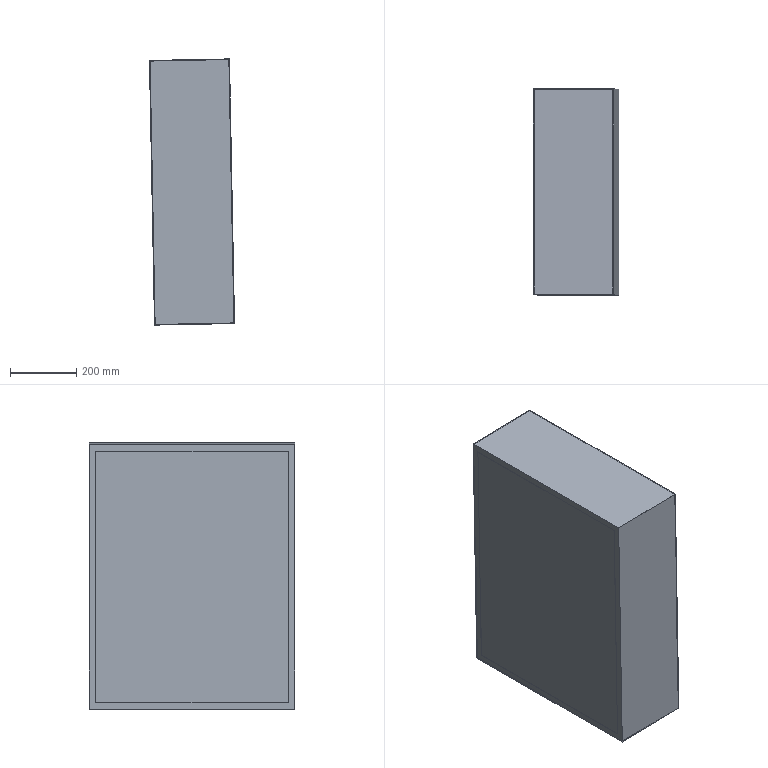Component | SolidWorks | PowerDistributionCabinet-1 | 2 solids | 22 faces | box 257.19 x 622 x 804.46 mm | volume 4667296 mm3 | plane 22 | material A3 Steel
build123d program:
from build123d import *

# Parameters (mm, degrees)
SKETCH1_W           = 800
SKETCH1_H           = 622
SKETCH1_W_2         = 796
SKETCH1_H_2         = 618
EXTRUDE_THIN1_DEPTH = 120
SKETCH2_W           = 800
SKETCH2_H           = 622
BOSS_EXTRUDE1_DEPTH = 2
SKETCH3_W           = 800
SKETCH3_H           = 622
SKETCH3_W_2         = 760
SKETCH3_H_2         = 582
BOSS_EXTRUDE2_DEPTH = 2
SKETCH4_W           = 760
SKETCH4_H           = 582
BOSS_EXTRUDE3_DEPTH = 5


with BuildPart() as part:
    # Sketch1 → Extrude-Thin1 (new, symmetric)
    with BuildSketch(Plane.XY):
        Rectangle(SKETCH1_W, SKETCH1_H)
        Rectangle(SKETCH1_W_2, SKETCH1_H_2, mode=Mode.SUBTRACT)
    extrude(amount=EXTRUDE_THIN1_DEPTH, both=True)

    # Sketch2 → Boss-Extrude1 (add)
    with BuildSketch(Plane.XY.offset(120)):
        Rectangle(SKETCH2_W, SKETCH2_H)
    extrude(amount=-BOSS_EXTRUDE1_DEPTH)

    # Sketch3 → Boss-Extrude2 (add)
    with BuildSketch(Plane(origin=(0, 0, -120), x_dir=(-1, 0, 0), z_dir=(0, 0, -1))):
        Rectangle(SKETCH3_W, SKETCH3_H)
        Rectangle(SKETCH3_W_2, SKETCH3_H_2, mode=Mode.SUBTRACT)
    extrude(amount=BOSS_EXTRUDE2_DEPTH)


with BuildPart() as body_2:
    # Sketch4 → Boss-Extrude3 (new body)
    with BuildSketch(Plane(origin=(0, 0, -122), x_dir=(-1, 0, 0), z_dir=(0, 0, -1))):
        Rectangle(SKETCH4_W, SKETCH4_H)
    extrude(amount=-BOSS_EXTRUDE3_DEPTH)


solid = Compound([part.part, body_2.part])

# Placed as in the assembly
solid = solid.moved(Location((-712.476, -1999.522, 1921.522), (0, 88.909, 180)))
STEP:
#1=CARTESIAN_POINT('',(-33.137,-90.178,90.517));
#2=VERTEX_POINT('',#1);
#3=CARTESIAN_POINT('',(-33.137,-67.265,90.517));
#4=VERTEX_POINT('',#3);
#5=CARTESIAN_POINT('',(-33.137,-90.178,90.517));
#6=DIRECTION('',(-0.,1.,-0.));
#7=VECTOR('',#6,39.37);
#8=LINE('',#5,#7);
#9=EDGE_CURVE('',#2,#4,#8,.T.);
#10=ORIENTED_EDGE('',*,*,#9,.F.);
#11=CARTESIAN_POINT('',(-32.941,-90.178,90.521));
#12=VERTEX_POINT('',#11);
#13=CARTESIAN_POINT('',(-32.941,-90.178,90.521));
#14=DIRECTION('',(-0.9998,-0.,-0.01904));
#15=VECTOR('',#14,39.37);
#16=LINE('',#13,#15);
#17=EDGE_CURVE('',#12,#2,#16,.T.);
#18=ORIENTED_EDGE('',*,*,#17,.F.);
#19=CARTESIAN_POINT('',(-32.941,-67.265,90.521));
#20=VERTEX_POINT('',#19);
#21=CARTESIAN_POINT('',(-32.941,-90.178,90.521));
#22=DIRECTION('',(-0.,1.,-0.));
#23=VECTOR('',#22,39.37);
#24=LINE('',#21,#23);
#25=EDGE_CURVE('',#12,#20,#24,.T.);
#26=ORIENTED_EDGE('',*,*,#25,.T.);
#27=CARTESIAN_POINT('',(-32.941,-67.265,90.521));
#28=DIRECTION('',(-0.9998,-0.,-0.01904));
#29=VECTOR('',#28,39.37);
#30=LINE('',#27,#29);
#31=EDGE_CURVE('',#20,#4,#30,.T.);
#32=ORIENTED_EDGE('',*,*,#31,.T.);
#33=EDGE_LOOP('',(#10,#18,#26,#32));
#34=FACE_OUTER_BOUND('',#33,.T.);
#35=CARTESIAN_POINT('',(-32.941,-90.178,90.521));
#36=DIRECTION('',(-0.01904,0.,0.9998));
#37=DIRECTION('',(0.9998,0.,0.01904));
#38=AXIS2_PLACEMENT_3D('',#35,#36,#37);
#39=PLANE('',#38);
#40=ADVANCED_FACE('',(#34),#39,.T.);
#41=CARTESIAN_POINT('',(-32.568,-90.178,60.601));
#42=VERTEX_POINT('',#41);
#43=CARTESIAN_POINT('',(-32.568,-90.178,60.601));
#44=DIRECTION('',(-0.01904,0.,0.9998));
#45=VECTOR('',#44,39.37);
#46=LINE('',#43,#45);
#47=EDGE_CURVE('',#42,#2,#46,.T.);
#48=ORIENTED_EDGE('',*,*,#47,.F.);
#49=CARTESIAN_POINT('',(-32.371,-90.178,60.605));
#50=VERTEX_POINT('',#49);
#51=CARTESIAN_POINT('',(-32.371,-90.178,60.605));
#52=DIRECTION('',(-0.9998,-0.,-0.01904));
#53=VECTOR('',#52,39.37);
#54=LINE('',#51,#53);
#55=EDGE_CURVE('',#50,#42,#54,.T.);
#56=ORIENTED_EDGE('',*,*,#55,.F.);
#57=CARTESIAN_POINT('',(-32.371,-90.178,60.605));
#58=DIRECTION('',(-0.01904,0.,0.9998));
#59=VECTOR('',#58,39.37);
#60=LINE('',#57,#59);
#61=EDGE_CURVE('',#50,#12,#60,.T.);
#62=ORIENTED_EDGE('',*,*,#61,.T.);
#63=ORIENTED_EDGE('',*,*,#17,.T.);
#64=EDGE_LOOP('',(#48,#56,#62,#63));
#65=FACE_OUTER_BOUND('',#64,.T.);
#66=CARTESIAN_POINT('',(-32.371,-90.178,60.605));
#67=DIRECTION('',(0.,-1.,0.));
#68=DIRECTION('',(-0.9998,-0.,-0.01904));
#69=AXIS2_PLACEMENT_3D('',#66,#67,#68);
#70=PLANE('',#69);
#71=ADVANCED_FACE('',(#65),#70,.T.);
#72=CARTESIAN_POINT('',(-32.568,-67.265,60.601));
#73=VERTEX_POINT('',#72);
#74=CARTESIAN_POINT('',(-32.568,-90.178,60.601));
#75=DIRECTION('',(0.,-1.,0.));
#76=VECTOR('',#75,39.37);
#77=LINE('',#74,#76);
#78=EDGE_CURVE('',#73,#42,#77,.T.);
#79=ORIENTED_EDGE('',*,*,#78,.F.);
#80=CARTESIAN_POINT('',(-32.371,-67.265,60.605));
#81=VERTEX_POINT('',#80);
#82=CARTESIAN_POINT('',(-32.371,-67.265,60.605));
#83=DIRECTION('',(-0.9998,-0.,-0.01904));
#84=VECTOR('',#83,39.37);
#85=LINE('',#82,#84);
#86=EDGE_CURVE('',#81,#73,#85,.T.);
#87=ORIENTED_EDGE('',*,*,#86,.F.);
#88=CARTESIAN_POINT('',(-32.371,-90.178,60.605));
#89=DIRECTION('',(0.,-1.,0.));
#90=VECTOR('',#89,39.37);
#91=LINE('',#88,#90);
#92=EDGE_CURVE('',#81,#50,#91,.T.);
#93=ORIENTED_EDGE('',*,*,#92,.T.);
#94=ORIENTED_EDGE('',*,*,#55,.T.);
#95=EDGE_LOOP('',(#79,#87,#93,#94));
#96=FACE_OUTER_BOUND('',#95,.T.);
#97=CARTESIAN_POINT('',(-32.371,-90.178,60.605));
#98=DIRECTION('',(0.01904,-0.,-0.9998));
#99=DIRECTION('',(-0.9998,-0.,-0.01904));
#100=AXIS2_PLACEMENT_3D('',#97,#98,#99);
#101=PLANE('',#100);
#102=ADVANCED_FACE('',(#96),#101,.T.);
#103=CARTESIAN_POINT('',(-32.568,-67.265,60.601));
#104=DIRECTION('',(0.01904,-0.,-0.9998));
#105=VECTOR('',#104,39.37);
#106=LINE('',#103,#105);
#107=EDGE_CURVE('',#4,#73,#106,.T.);
#108=ORIENTED_EDGE('',*,*,#107,.F.);
#109=ORIENTED_EDGE('',*,*,#31,.F.);
#110=CARTESIAN_POINT('',(-32.371,-67.265,60.605));
#111=DIRECTION('',(0.01904,-0.,-0.9998));
#112=VECTOR('',#111,39.37);
#113=LINE('',#110,#112);
#114=EDGE_CURVE('',#20,#81,#113,.T.);
#115=ORIENTED_EDGE('',*,*,#114,.T.);
#116=ORIENTED_EDGE('',*,*,#86,.T.);
#117=EDGE_LOOP('',(#108,#109,#115,#116));
#118=FACE_OUTER_BOUND('',#117,.T.);
#119=CARTESIAN_POINT('',(-32.371,-67.265,60.605));
#120=DIRECTION('',(-0.,1.,-0.));
#121=DIRECTION('',(0.9998,0.,0.01904));
#122=AXIS2_PLACEMENT_3D('',#119,#120,#121);
#123=PLANE('',#122);
#124=ADVANCED_FACE('',(#118),#123,.T.);
#125=ORIENTED_EDGE('',*,*,#25,.F.);
#126=ORIENTED_EDGE('',*,*,#61,.F.);
#127=ORIENTED_EDGE('',*,*,#92,.F.);
#128=ORIENTED_EDGE('',*,*,#114,.F.);
#129=EDGE_LOOP('',(#125,#126,#127,#128));
#130=FACE_OUTER_BOUND('',#129,.T.);
#131=CARTESIAN_POINT('',(-32.656,-78.721,75.563));
#132=DIRECTION('',(0.9998,0.,0.01904));
#133=DIRECTION('',(0.01904,-0.,-0.9998));
#134=AXIS2_PLACEMENT_3D('',#131,#132,#133);
#135=PLANE('',#134);
#136=ADVANCED_FACE('',(#130),#135,.T.);
#137=ORIENTED_EDGE('',*,*,#9,.T.);
#138=ORIENTED_EDGE('',*,*,#107,.T.);
#139=ORIENTED_EDGE('',*,*,#78,.T.);
#140=ORIENTED_EDGE('',*,*,#47,.T.);
#141=EDGE_LOOP('',(#137,#138,#139,#140));
#142=FACE_OUTER_BOUND('',#141,.T.);
#143=CARTESIAN_POINT('',(-32.853,-78.721,75.559));
#144=DIRECTION('',(0.9998,0.,0.01904));
#145=DIRECTION('',(0.01904,-0.,-0.9998));
#146=AXIS2_PLACEMENT_3D('',#143,#144,#145);
#147=PLANE('',#146);
#148=ADVANCED_FACE('',(#142),#147,.F.);
#149=CLOSED_SHELL('',(#40,#71,#102,#124,#136,#148));
#150=MANIFOLD_SOLID_BREP('',#149);
#151=CARTESIAN_POINT('',(-23.107,-90.887,60.073));
#152=VERTEX_POINT('',#151);
#153=CARTESIAN_POINT('',(-32.475,-90.887,59.894));
#154=VERTEX_POINT('',#153);
#155=CARTESIAN_POINT('',(-23.028,-90.887,60.074));
#156=DIRECTION('',(-0.9998,-0.,-0.01904));
#157=VECTOR('',#156,39.37);
#158=LINE('',#155,#157);
#159=EDGE_CURVE('',#152,#154,#158,.T.);
#160=ORIENTED_EDGE('',*,*,#159,.F.);
#161=CARTESIAN_POINT('',(-23.107,-66.556,60.073));
#162=VERTEX_POINT('',#161);
#163=CARTESIAN_POINT('',(-23.107,-78.721,60.073));
#164=DIRECTION('',(-0.,1.,-0.));
#165=VECTOR('',#164,39.37);
#166=LINE('',#163,#165);
#167=EDGE_CURVE('',#152,#162,#166,.T.);
#168=ORIENTED_EDGE('',*,*,#167,.T.);
#169=CARTESIAN_POINT('',(-32.475,-66.556,59.894));
#170=VERTEX_POINT('',#169);
#171=CARTESIAN_POINT('',(-23.028,-66.556,60.074));
#172=DIRECTION('',(-0.9998,-0.,-0.01904));
#173=VECTOR('',#172,39.37);
#174=LINE('',#171,#173);
#175=EDGE_CURVE('',#162,#170,#174,.T.);
#176=ORIENTED_EDGE('',*,*,#175,.T.);
#177=CARTESIAN_POINT('',(-32.475,-78.721,59.894));
#178=DIRECTION('',(-0.,1.,-0.));
#179=VECTOR('',#178,39.37);
#180=LINE('',#177,#179);
#181=EDGE_CURVE('',#154,#170,#180,.T.);
#182=ORIENTED_EDGE('',*,*,#181,.F.);
#183=EDGE_LOOP('',(#160,#168,#176,#182));
#184=FACE_OUTER_BOUND('',#183,.T.);
#185=CARTESIAN_POINT('',(-23.028,-78.721,60.074));
#186=DIRECTION('',(-0.01904,0.,0.9998));
#187=DIRECTION('',(0.9998,0.,0.01904));
#188=AXIS2_PLACEMENT_3D('',#185,#186,#187);
#189=PLANE('',#188);
#190=ADVANCED_FACE('',(#184),#189,.T.);
#191=ORIENTED_EDGE('',*,*,#175,.F.);
#192=CARTESIAN_POINT('',(-23.704,-66.556,91.405));
#193=VERTEX_POINT('',#192);
#194=CARTESIAN_POINT('',(-23.405,-66.556,75.739));
#195=DIRECTION('',(-0.01904,0.,0.9998));
#196=VECTOR('',#195,39.37);
#197=LINE('',#194,#196);
#198=EDGE_CURVE('',#162,#193,#197,.T.);
#199=ORIENTED_EDGE('',*,*,#198,.T.);
#200=CARTESIAN_POINT('',(-33.072,-66.556,91.227));
#201=VERTEX_POINT('',#200);
#202=CARTESIAN_POINT('',(-23.625,-66.556,91.407));
#203=DIRECTION('',(-0.9998,-0.,-0.01904));
#204=VECTOR('',#203,39.37);
#205=LINE('',#202,#204);
#206=EDGE_CURVE('',#193,#201,#205,.T.);
#207=ORIENTED_EDGE('',*,*,#206,.T.);
#208=CARTESIAN_POINT('',(-32.774,-66.556,75.561));
#209=DIRECTION('',(-0.01904,0.,0.9998));
#210=VECTOR('',#209,39.37);
#211=LINE('',#208,#210);
#212=EDGE_CURVE('',#170,#201,#211,.T.);
#213=ORIENTED_EDGE('',*,*,#212,.F.);
#214=EDGE_LOOP('',(#191,#199,#207,#213));
#215=FACE_OUTER_BOUND('',#214,.T.);
#216=CARTESIAN_POINT('',(-23.327,-66.556,75.74));
#217=DIRECTION('',(0.,-1.,0.));
#218=DIRECTION('',(-0.9998,-0.,-0.01904));
#219=AXIS2_PLACEMENT_3D('',#216,#217,#218);
#220=PLANE('',#219);
#221=ADVANCED_FACE('',(#215),#220,.T.);
#222=ORIENTED_EDGE('',*,*,#206,.F.);
#223=CARTESIAN_POINT('',(-23.704,-90.887,91.405));
#224=VERTEX_POINT('',#223);
#225=CARTESIAN_POINT('',(-23.704,-78.721,91.405));
#226=DIRECTION('',(0.,-1.,0.));
#227=VECTOR('',#226,39.37);
#228=LINE('',#225,#227);
#229=EDGE_CURVE('',#193,#224,#228,.T.);
#230=ORIENTED_EDGE('',*,*,#229,.T.);
#231=CARTESIAN_POINT('',(-33.072,-90.887,91.227));
#232=VERTEX_POINT('',#231);
#233=CARTESIAN_POINT('',(-23.625,-90.887,91.407));
#234=DIRECTION('',(-0.9998,-0.,-0.01904));
#235=VECTOR('',#234,39.37);
#236=LINE('',#233,#235);
#237=EDGE_CURVE('',#224,#232,#236,.T.);
#238=ORIENTED_EDGE('',*,*,#237,.T.);
#239=CARTESIAN_POINT('',(-33.072,-78.721,91.227));
#240=DIRECTION('',(0.,-1.,0.));
#241=VECTOR('',#240,39.37);
#242=LINE('',#239,#241);
#243=EDGE_CURVE('',#201,#232,#242,.T.);
#244=ORIENTED_EDGE('',*,*,#243,.F.);
#245=EDGE_LOOP('',(#222,#230,#238,#244));
#246=FACE_OUTER_BOUND('',#245,.T.);
#247=CARTESIAN_POINT('',(-23.625,-78.721,91.407));
#248=DIRECTION('',(0.01904,-0.,-0.9998));
#249=DIRECTION('',(-0.9998,-0.,-0.01904));
#250=AXIS2_PLACEMENT_3D('',#247,#248,#249);
#251=PLANE('',#250);
#252=ADVANCED_FACE('',(#246),#251,.T.);
#253=ORIENTED_EDGE('',*,*,#237,.F.);
#254=CARTESIAN_POINT('',(-23.405,-90.887,75.739));
#255=DIRECTION('',(0.01904,-0.,-0.9998));
#256=VECTOR('',#255,39.37);
#257=LINE('',#254,#256);
#258=EDGE_CURVE('',#224,#152,#257,.T.);
#259=ORIENTED_EDGE('',*,*,#258,.T.);
#260=ORIENTED_EDGE('',*,*,#159,.T.);
#261=CARTESIAN_POINT('',(-32.774,-90.887,75.561));
#262=DIRECTION('',(0.01904,-0.,-0.9998));
#263=VECTOR('',#262,39.37);
#264=LINE('',#261,#263);
#265=EDGE_CURVE('',#232,#154,#264,.T.);
#266=ORIENTED_EDGE('',*,*,#265,.F.);
#267=EDGE_LOOP('',(#253,#259,#260,#266));
#268=FACE_OUTER_BOUND('',#267,.T.);
#269=CARTESIAN_POINT('',(-23.327,-90.887,75.74));
#270=DIRECTION('',(-0.,1.,-0.));
#271=DIRECTION('',(0.9998,0.,0.01904));
#272=AXIS2_PLACEMENT_3D('',#269,#270,#271);
#273=PLANE('',#272);
#274=ADVANCED_FACE('',(#268),#273,.T.);
#275=ORIENTED_EDGE('',*,*,#167,.F.);
#276=ORIENTED_EDGE('',*,*,#258,.F.);
#277=ORIENTED_EDGE('',*,*,#229,.F.);
#278=ORIENTED_EDGE('',*,*,#198,.F.);
#279=EDGE_LOOP('',(#275,#276,#277,#278));
#280=FACE_OUTER_BOUND('',#279,.T.);
#281=CARTESIAN_POINT('',(-23.405,-78.721,75.739));
#282=DIRECTION('',(0.9998,0.,0.01904));
#283=DIRECTION('',(0.01904,-0.,-0.9998));
#284=AXIS2_PLACEMENT_3D('',#281,#282,#283);
#285=PLANE('',#284);
#286=ADVANCED_FACE('',(#280),#285,.F.);
#287=CARTESIAN_POINT('',(-33.152,-66.477,91.304));
#288=VERTEX_POINT('',#287);
#289=CARTESIAN_POINT('',(-32.553,-66.477,59.814));
#290=VERTEX_POINT('',#289);
#291=CARTESIAN_POINT('',(-33.152,-66.477,91.304));
#292=DIRECTION('',(0.01904,-0.,-0.9998));
#293=VECTOR('',#292,39.37);
#294=LINE('',#291,#293);
#295=EDGE_CURVE('',#288,#290,#294,.T.);
#296=ORIENTED_EDGE('',*,*,#295,.T.);
#297=CARTESIAN_POINT('',(-32.553,-90.965,59.814));
#298=VERTEX_POINT('',#297);
#299=CARTESIAN_POINT('',(-32.553,-66.477,59.814));
#300=DIRECTION('',(0.,-1.,0.));
#301=VECTOR('',#300,39.37);
#302=LINE('',#299,#301);
#303=EDGE_CURVE('',#290,#298,#302,.T.);
#304=ORIENTED_EDGE('',*,*,#303,.T.);
#305=CARTESIAN_POINT('',(-33.152,-90.965,91.304));
#306=VERTEX_POINT('',#305);
#307=CARTESIAN_POINT('',(-32.553,-90.965,59.814));
#308=DIRECTION('',(-0.01904,0.,0.9998));
#309=VECTOR('',#308,39.37);
#310=LINE('',#307,#309);
#311=EDGE_CURVE('',#298,#306,#310,.T.);
#312=ORIENTED_EDGE('',*,*,#311,.T.);
#313=CARTESIAN_POINT('',(-33.152,-90.965,91.304));
#314=DIRECTION('',(-0.,1.,-0.));
#315=VECTOR('',#314,39.37);
#316=LINE('',#313,#315);
#317=EDGE_CURVE('',#306,#288,#316,.T.);
#318=ORIENTED_EDGE('',*,*,#317,.T.);
#319=EDGE_LOOP('',(#296,#304,#312,#318));
#320=FACE_OUTER_BOUND('',#319,.T.);
#321=CARTESIAN_POINT('',(-33.137,-67.265,90.517));
#322=VERTEX_POINT('',#321);
#323=CARTESIAN_POINT('',(-32.568,-67.265,60.601));
#324=VERTEX_POINT('',#323);
#325=CARTESIAN_POINT('',(-32.568,-67.265,60.601));
#326=DIRECTION('',(0.01904,-0.,-0.9998));
#327=VECTOR('',#326,39.37);
#328=LINE('',#325,#327);
#329=EDGE_CURVE('',#322,#324,#328,.T.);
#330=ORIENTED_EDGE('',*,*,#329,.F.);
#331=CARTESIAN_POINT('',(-33.137,-90.178,90.517));
#332=VERTEX_POINT('',#331);
#333=CARTESIAN_POINT('',(-33.137,-90.178,90.517));
#334=DIRECTION('',(-0.,1.,-0.));
#335=VECTOR('',#334,39.37);
#336=LINE('',#333,#335);
#337=EDGE_CURVE('',#332,#322,#336,.T.);
#338=ORIENTED_EDGE('',*,*,#337,.F.);
#339=CARTESIAN_POINT('',(-32.568,-90.178,60.601));
#340=VERTEX_POINT('',#339);
#341=CARTESIAN_POINT('',(-32.568,-90.178,60.601));
#342=DIRECTION('',(-0.01904,0.,0.9998));
#343=VECTOR('',#342,39.37);
#344=LINE('',#341,#343);
#345=EDGE_CURVE('',#340,#332,#344,.T.);
#346=ORIENTED_EDGE('',*,*,#345,.F.);
#347=CARTESIAN_POINT('',(-32.568,-90.178,60.601));
#348=DIRECTION('',(0.,-1.,0.));
#349=VECTOR('',#348,39.37);
#350=LINE('',#347,#349);
#351=EDGE_CURVE('',#324,#340,#350,.T.);
#352=ORIENTED_EDGE('',*,*,#351,.F.);
#353=EDGE_LOOP('',(#330,#338,#346,#352));
#354=FACE_BOUND('',#353,.T.);
#355=CARTESIAN_POINT('',(-32.853,-78.721,75.559));
#356=DIRECTION('',(-0.9998,-0.,-0.01904));
#357=DIRECTION('',(-0.01904,0.,0.9998));
#358=AXIS2_PLACEMENT_3D('',#355,#356,#357);
#359=PLANE('',#358);
#360=ADVANCED_FACE('',(#320,#354),#359,.T.);
#361=ORIENTED_EDGE('',*,*,#181,.T.);
#362=ORIENTED_EDGE('',*,*,#212,.T.);
#363=ORIENTED_EDGE('',*,*,#243,.T.);
#364=ORIENTED_EDGE('',*,*,#265,.T.);
#365=EDGE_LOOP('',(#361,#362,#363,#364));
#366=FACE_OUTER_BOUND('',#365,.T.);
#367=CARTESIAN_POINT('',(-33.059,-90.178,90.518));
#368=VERTEX_POINT('',#367);
#369=CARTESIAN_POINT('',(-33.059,-67.265,90.518));
#370=VERTEX_POINT('',#369);
#371=CARTESIAN_POINT('',(-33.059,-90.178,90.518));
#372=DIRECTION('',(-0.,1.,-0.));
#373=VECTOR('',#372,39.37);
#374=LINE('',#371,#373);
#375=EDGE_CURVE('',#368,#370,#374,.T.);
#376=ORIENTED_EDGE('',*,*,#375,.T.);
#377=CARTESIAN_POINT('',(-32.489,-67.265,60.603));
#378=VERTEX_POINT('',#377);
#379=CARTESIAN_POINT('',(-32.489,-67.265,60.603));
#380=DIRECTION('',(0.01904,-0.,-0.9998));
#381=VECTOR('',#380,39.37);
#382=LINE('',#379,#381);
#383=EDGE_CURVE('',#370,#378,#382,.T.);
#384=ORIENTED_EDGE('',*,*,#383,.T.);
#385=CARTESIAN_POINT('',(-32.489,-90.178,60.603));
#386=VERTEX_POINT('',#385);
#387=CARTESIAN_POINT('',(-32.489,-90.178,60.603));
#388=DIRECTION('',(0.,-1.,0.));
#389=VECTOR('',#388,39.37);
#390=LINE('',#387,#389);
#391=EDGE_CURVE('',#378,#386,#390,.T.);
#392=ORIENTED_EDGE('',*,*,#391,.T.);
#393=CARTESIAN_POINT('',(-32.489,-90.178,60.603));
#394=DIRECTION('',(-0.01904,0.,0.9998));
#395=VECTOR('',#394,39.37);
#396=LINE('',#393,#395);
#397=EDGE_CURVE('',#386,#368,#396,.T.);
#398=ORIENTED_EDGE('',*,*,#397,.T.);
#399=EDGE_LOOP('',(#376,#384,#392,#398));
#400=FACE_BOUND('',#399,.T.);
#401=CARTESIAN_POINT('',(-32.774,-78.721,75.561));
#402=DIRECTION('',(-0.9998,-0.,-0.01904));
#403=DIRECTION('',(-0.01904,0.,0.9998));
#404=AXIS2_PLACEMENT_3D('',#401,#402,#403);
#405=PLANE('',#404);
#406=ADVANCED_FACE('',(#366,#400),#405,.F.);
#407=ORIENTED_EDGE('',*,*,#375,.F.);
#408=CARTESIAN_POINT('',(-33.137,-90.178,90.517));
#409=DIRECTION('',(0.9998,0.,0.01904));
#410=VECTOR('',#409,39.37);
#411=LINE('',#408,#410);
#412=EDGE_CURVE('',#332,#368,#411,.T.);
#413=ORIENTED_EDGE('',*,*,#412,.F.);
#414=ORIENTED_EDGE('',*,*,#337,.T.);
#415=CARTESIAN_POINT('',(-33.137,-67.265,90.517));
#416=DIRECTION('',(0.9998,0.,0.01904));
#417=VECTOR('',#416,39.37);
#418=LINE('',#415,#417);
#419=EDGE_CURVE('',#322,#370,#418,.T.);
#420=ORIENTED_EDGE('',*,*,#419,.T.);
#421=EDGE_LOOP('',(#407,#413,#414,#420));
#422=FACE_OUTER_BOUND('',#421,.T.);
#423=CARTESIAN_POINT('',(-33.137,-90.178,90.517));
#424=DIRECTION('',(0.01904,-0.,-0.9998));
#425=DIRECTION('',(-0.9998,-0.,-0.01904));
#426=AXIS2_PLACEMENT_3D('',#423,#424,#425);
#427=PLANE('',#426);
#428=ADVANCED_FACE('',(#422),#427,.T.);
#429=ORIENTED_EDGE('',*,*,#383,.F.);
#430=ORIENTED_EDGE('',*,*,#419,.F.);
#431=ORIENTED_EDGE('',*,*,#329,.T.);
#432=CARTESIAN_POINT('',(-32.568,-67.265,60.601));
#433=DIRECTION('',(0.9998,0.,0.01904));
#434=VECTOR('',#433,39.37);
#435=LINE('',#432,#434);
#436=EDGE_CURVE('',#324,#378,#435,.T.);
#437=ORIENTED_EDGE('',*,*,#436,.T.);
#438=EDGE_LOOP('',(#429,#430,#431,#437));
#439=FACE_OUTER_BOUND('',#438,.T.);
#440=CARTESIAN_POINT('',(-32.568,-67.265,60.601));
#441=DIRECTION('',(0.,-1.,0.));
#442=DIRECTION('',(-0.9998,-0.,-0.01904));
#443=AXIS2_PLACEMENT_3D('',#440,#441,#442);
#444=PLANE('',#443);
#445=ADVANCED_FACE('',(#439),#444,.T.);
#446=ORIENTED_EDGE('',*,*,#391,.F.);
#447=ORIENTED_EDGE('',*,*,#436,.F.);
#448=ORIENTED_EDGE('',*,*,#351,.T.);
#449=CARTESIAN_POINT('',(-32.568,-90.178,60.601));
#450=DIRECTION('',(0.9998,0.,0.01904));
#451=VECTOR('',#450,39.37);
#452=LINE('',#449,#451);
#453=EDGE_CURVE('',#340,#386,#452,.T.);
#454=ORIENTED_EDGE('',*,*,#453,.T.);
#455=EDGE_LOOP('',(#446,#447,#448,#454));
#456=FACE_OUTER_BOUND('',#455,.T.);
#457=CARTESIAN_POINT('',(-32.568,-90.178,60.601));
#458=DIRECTION('',(-0.01904,0.,0.9998));
#459=DIRECTION('',(0.9998,0.,0.01904));
#460=AXIS2_PLACEMENT_3D('',#457,#458,#459);
#461=PLANE('',#460);
#462=ADVANCED_FACE('',(#456),#461,.T.);
#463=ORIENTED_EDGE('',*,*,#397,.F.);
#464=ORIENTED_EDGE('',*,*,#453,.F.);
#465=ORIENTED_EDGE('',*,*,#345,.T.);
#466=ORIENTED_EDGE('',*,*,#412,.T.);
#467=EDGE_LOOP('',(#463,#464,#465,#466));
#468=FACE_OUTER_BOUND('',#467,.T.);
#469=CARTESIAN_POINT('',(-32.568,-90.178,60.601));
#470=DIRECTION('',(-0.,1.,-0.));
#471=DIRECTION('',(0.9998,0.,0.01904));
#472=AXIS2_PLACEMENT_3D('',#469,#470,#471);
#473=PLANE('',#472);
#474=ADVANCED_FACE('',(#468),#473,.T.);
#475=CARTESIAN_POINT('',(-23.027,-90.965,59.995));
#476=VERTEX_POINT('',#475);
#477=CARTESIAN_POINT('',(-23.027,-66.477,59.995));
#478=VERTEX_POINT('',#477);
#479=CARTESIAN_POINT('',(-23.027,-78.721,59.995));
#480=DIRECTION('',(-0.,1.,-0.));
#481=VECTOR('',#480,39.37);
#482=LINE('',#479,#481);
#483=EDGE_CURVE('',#476,#478,#482,.T.);
#484=ORIENTED_EDGE('',*,*,#483,.T.);
#485=CARTESIAN_POINT('',(-23.627,-66.477,91.486));
#486=VERTEX_POINT('',#485);
#487=CARTESIAN_POINT('',(-23.327,-66.477,75.74));
#488=DIRECTION('',(-0.01904,0.,0.9998));
#489=VECTOR('',#488,39.37);
#490=LINE('',#487,#489);
#491=EDGE_CURVE('',#478,#486,#490,.T.);
#492=ORIENTED_EDGE('',*,*,#491,.T.);
#493=CARTESIAN_POINT('',(-23.627,-90.965,91.486));
#494=VERTEX_POINT('',#493);
#495=CARTESIAN_POINT('',(-23.627,-78.721,91.486));
#496=DIRECTION('',(0.,-1.,0.));
#497=VECTOR('',#496,39.37);
#498=LINE('',#495,#497);
#499=EDGE_CURVE('',#486,#494,#498,.T.);
#500=ORIENTED_EDGE('',*,*,#499,.T.);
#501=CARTESIAN_POINT('',(-23.327,-90.965,75.74));
#502=DIRECTION('',(0.01904,-0.,-0.9998));
#503=VECTOR('',#502,39.37);
#504=LINE('',#501,#503);
#505=EDGE_CURVE('',#494,#476,#504,.T.);
#506=ORIENTED_EDGE('',*,*,#505,.T.);
#507=EDGE_LOOP('',(#484,#492,#500,#506));
#508=FACE_OUTER_BOUND('',#507,.T.);
#509=CARTESIAN_POINT('',(-23.327,-78.721,75.74));
#510=DIRECTION('',(0.9998,0.,0.01904));
#511=DIRECTION('',(0.01904,-0.,-0.9998));
#512=AXIS2_PLACEMENT_3D('',#509,#510,#511);
#513=PLANE('',#512);
#514=ADVANCED_FACE('',(#508),#513,.T.);
#515=CARTESIAN_POINT('',(-23.627,-90.965,91.486));
#516=DIRECTION('',(-0.9998,-0.,-0.01904));
#517=VECTOR('',#516,39.37);
#518=LINE('',#515,#517);
#519=EDGE_CURVE('',#494,#306,#518,.T.);
#520=ORIENTED_EDGE('',*,*,#519,.T.);
#521=ORIENTED_EDGE('',*,*,#311,.F.);
#522=CARTESIAN_POINT('',(-23.027,-90.965,59.995));
#523=DIRECTION('',(-0.9998,-0.,-0.01904));
#524=VECTOR('',#523,39.37);
#525=LINE('',#522,#524);
#526=EDGE_CURVE('',#476,#298,#525,.T.);
#527=ORIENTED_EDGE('',*,*,#526,.F.);
#528=ORIENTED_EDGE('',*,*,#505,.F.);
#529=EDGE_LOOP('',(#520,#521,#527,#528));
#530=FACE_OUTER_BOUND('',#529,.T.);
#531=CARTESIAN_POINT('',(-23.327,-90.965,75.74));
#532=DIRECTION('',(-0.,1.,-0.));
#533=DIRECTION('',(0.9998,0.,0.01904));
#534=AXIS2_PLACEMENT_3D('',#531,#532,#533);
#535=PLANE('',#534);
#536=ADVANCED_FACE('',(#530),#535,.F.);
#537=CARTESIAN_POINT('',(-23.627,-66.477,91.486));
#538=DIRECTION('',(-0.9998,-0.,-0.01904));
#539=VECTOR('',#538,39.37);
#540=LINE('',#537,#539);
#541=EDGE_CURVE('',#486,#288,#540,.T.);
#542=ORIENTED_EDGE('',*,*,#541,.T.);
#543=ORIENTED_EDGE('',*,*,#317,.F.);
#544=ORIENTED_EDGE('',*,*,#519,.F.);
#545=ORIENTED_EDGE('',*,*,#499,.F.);
#546=EDGE_LOOP('',(#542,#543,#544,#545));
#547=FACE_OUTER_BOUND('',#546,.T.);
#548=CARTESIAN_POINT('',(-23.627,-78.721,91.486));
#549=DIRECTION('',(0.01904,-0.,-0.9998));
#550=DIRECTION('',(-0.9998,-0.,-0.01904));
#551=AXIS2_PLACEMENT_3D('',#548,#549,#550);
#552=PLANE('',#551);
#553=ADVANCED_FACE('',(#547),#552,.F.);
#554=CARTESIAN_POINT('',(-23.027,-66.477,59.995));
#555=DIRECTION('',(-0.9998,-0.,-0.01904));
#556=VECTOR('',#555,39.37);
#557=LINE('',#554,#556);
#558=EDGE_CURVE('',#478,#290,#557,.T.);
#559=ORIENTED_EDGE('',*,*,#558,.T.);
#560=ORIENTED_EDGE('',*,*,#295,.F.);
#561=ORIENTED_EDGE('',*,*,#541,.F.);
#562=ORIENTED_EDGE('',*,*,#491,.F.);
#563=EDGE_LOOP('',(#559,#560,#561,#562));
#564=FACE_OUTER_BOUND('',#563,.T.);
#565=CARTESIAN_POINT('',(-23.327,-66.477,75.74));
#566=DIRECTION('',(0.,-1.,0.));
#567=DIRECTION('',(-0.9998,-0.,-0.01904));
#568=AXIS2_PLACEMENT_3D('',#565,#566,#567);
#569=PLANE('',#568);
#570=ADVANCED_FACE('',(#564),#569,.F.);
#571=ORIENTED_EDGE('',*,*,#526,.T.);
#572=ORIENTED_EDGE('',*,*,#303,.F.);
#573=ORIENTED_EDGE('',*,*,#558,.F.);
#574=ORIENTED_EDGE('',*,*,#483,.F.);
#575=EDGE_LOOP('',(#571,#572,#573,#574));
#576=FACE_OUTER_BOUND('',#575,.T.);
#577=CARTESIAN_POINT('',(-23.027,-78.721,59.995));
#578=DIRECTION('',(-0.01904,0.,0.9998));
#579=DIRECTION('',(0.9998,0.,0.01904));
#580=AXIS2_PLACEMENT_3D('',#577,#578,#579);
#581=PLANE('',#580);
#582=ADVANCED_FACE('',(#576),#581,.F.);
#583=CLOSED_SHELL('',(#190,#221,#252,#274,#286,#360,#406,#428,#445,#462,#474,#514,#536,#553,#570,#582));
#584=MANIFOLD_SOLID_BREP('',#583);
#585=CARTESIAN_POINT('',(0.,0.,0.));
#586=DIRECTION('',(0.,0.,1.));
#587=DIRECTION('',(1.,0.,0.));
#588=AXIS2_PLACEMENT_3D('',#585,#586,#587);
#589=(LENGTH_UNIT()NAMED_UNIT(*)SI_UNIT($,.METRE.));
#590=LENGTH_MEASURE_WITH_UNIT(LENGTH_MEASURE(0.0254),#589);
#591=DIMENSIONAL_EXPONENTS(1.,0.,0.,0.,0.,0.,0.);
#592=(CONVERSION_BASED_UNIT('',#590)LENGTH_UNIT()NAMED_UNIT(#591));
#593=UNCERTAINTY_MEASURE_WITH_UNIT(LENGTH_MEASURE(0.00001),#592,'','');
#594=(NAMED_UNIT(*)PLANE_ANGLE_UNIT()SI_UNIT($,.RADIAN.));
#595=(NAMED_UNIT(*)SI_UNIT($,.STERADIAN.)SOLID_ANGLE_UNIT());
#596=(GEOMETRIC_REPRESENTATION_CONTEXT(3)GLOBAL_UNCERTAINTY_ASSIGNED_CONTEXT((#593))GLOBAL_UNIT_ASSIGNED_CONTEXT((#592,#594,#595))REPRESENTATION_CONTEXT('',''));
#597=ADVANCED_BREP_SHAPE_REPRESENTATION('',(#150,#584,#588),#596);
#598=COLOUR_RGB('',0.7922,0.8196,0.9333);
#599=FILL_AREA_STYLE_COLOUR('',#598);
#600=FILL_AREA_STYLE('',(#599));
#601=SURFACE_STYLE_FILL_AREA(#600);
#602=SURFACE_SIDE_STYLE('',(#601));
#603=SURFACE_STYLE_USAGE(.BOTH.,#602);
#604=PRESENTATION_STYLE_ASSIGNMENT((#603));
#605=STYLED_ITEM('',(#604),#584);
#606=PRESENTATION_LAYER_ASSIGNMENT('','',(#605));
#607=COLOUR_RGB('',0.7922,0.8196,0.9333);
#608=FILL_AREA_STYLE_COLOUR('',#607);
#609=FILL_AREA_STYLE('',(#608));
#610=SURFACE_STYLE_FILL_AREA(#609);
#611=SURFACE_SIDE_STYLE('',(#610));
#612=SURFACE_STYLE_USAGE(.BOTH.,#611);
#613=PRESENTATION_STYLE_ASSIGNMENT((#612));
#614=STYLED_ITEM('',(#613),#150);
#615=PRESENTATION_LAYER_ASSIGNMENT('','',(#614));
#616=(LENGTH_UNIT()NAMED_UNIT(*)SI_UNIT($,.METRE.));
#617=LENGTH_MEASURE_WITH_UNIT(LENGTH_MEASURE(0.0254),#616);
#618=DIMENSIONAL_EXPONENTS(1.,0.,0.,0.,0.,0.,0.);
#619=(CONVERSION_BASED_UNIT('',#617)LENGTH_UNIT()NAMED_UNIT(#618));
#620=UNCERTAINTY_MEASURE_WITH_UNIT(LENGTH_MEASURE(0.00001),#619,'','');
#621=(NAMED_UNIT(*)PLANE_ANGLE_UNIT()SI_UNIT($,.RADIAN.));
#622=(NAMED_UNIT(*)SI_UNIT($,.STERADIAN.)SOLID_ANGLE_UNIT());
#623=(GEOMETRIC_REPRESENTATION_CONTEXT(3)GLOBAL_UNCERTAINTY_ASSIGNED_CONTEXT((#620))GLOBAL_UNIT_ASSIGNED_CONTEXT((#619,#621,#622))REPRESENTATION_CONTEXT('',''));
#624=MECHANICAL_DESIGN_GEOMETRIC_PRESENTATION_REPRESENTATION('',(#605),#623);
#625=(LENGTH_UNIT()NAMED_UNIT(*)SI_UNIT($,.METRE.));
#626=LENGTH_MEASURE_WITH_UNIT(LENGTH_MEASURE(0.0254),#625);
#627=DIMENSIONAL_EXPONENTS(1.,0.,0.,0.,0.,0.,0.);
#628=(CONVERSION_BASED_UNIT('',#626)LENGTH_UNIT()NAMED_UNIT(#627));
#629=UNCERTAINTY_MEASURE_WITH_UNIT(LENGTH_MEASURE(0.00001),#628,'','');
#630=(NAMED_UNIT(*)PLANE_ANGLE_UNIT()SI_UNIT($,.RADIAN.));
#631=(NAMED_UNIT(*)SI_UNIT($,.STERADIAN.)SOLID_ANGLE_UNIT());
#632=(GEOMETRIC_REPRESENTATION_CONTEXT(3)GLOBAL_UNCERTAINTY_ASSIGNED_CONTEXT((#629))GLOBAL_UNIT_ASSIGNED_CONTEXT((#628,#630,#631))REPRESENTATION_CONTEXT('',''));
#633=MECHANICAL_DESIGN_GEOMETRIC_PRESENTATION_REPRESENTATION('',(#614),#632);